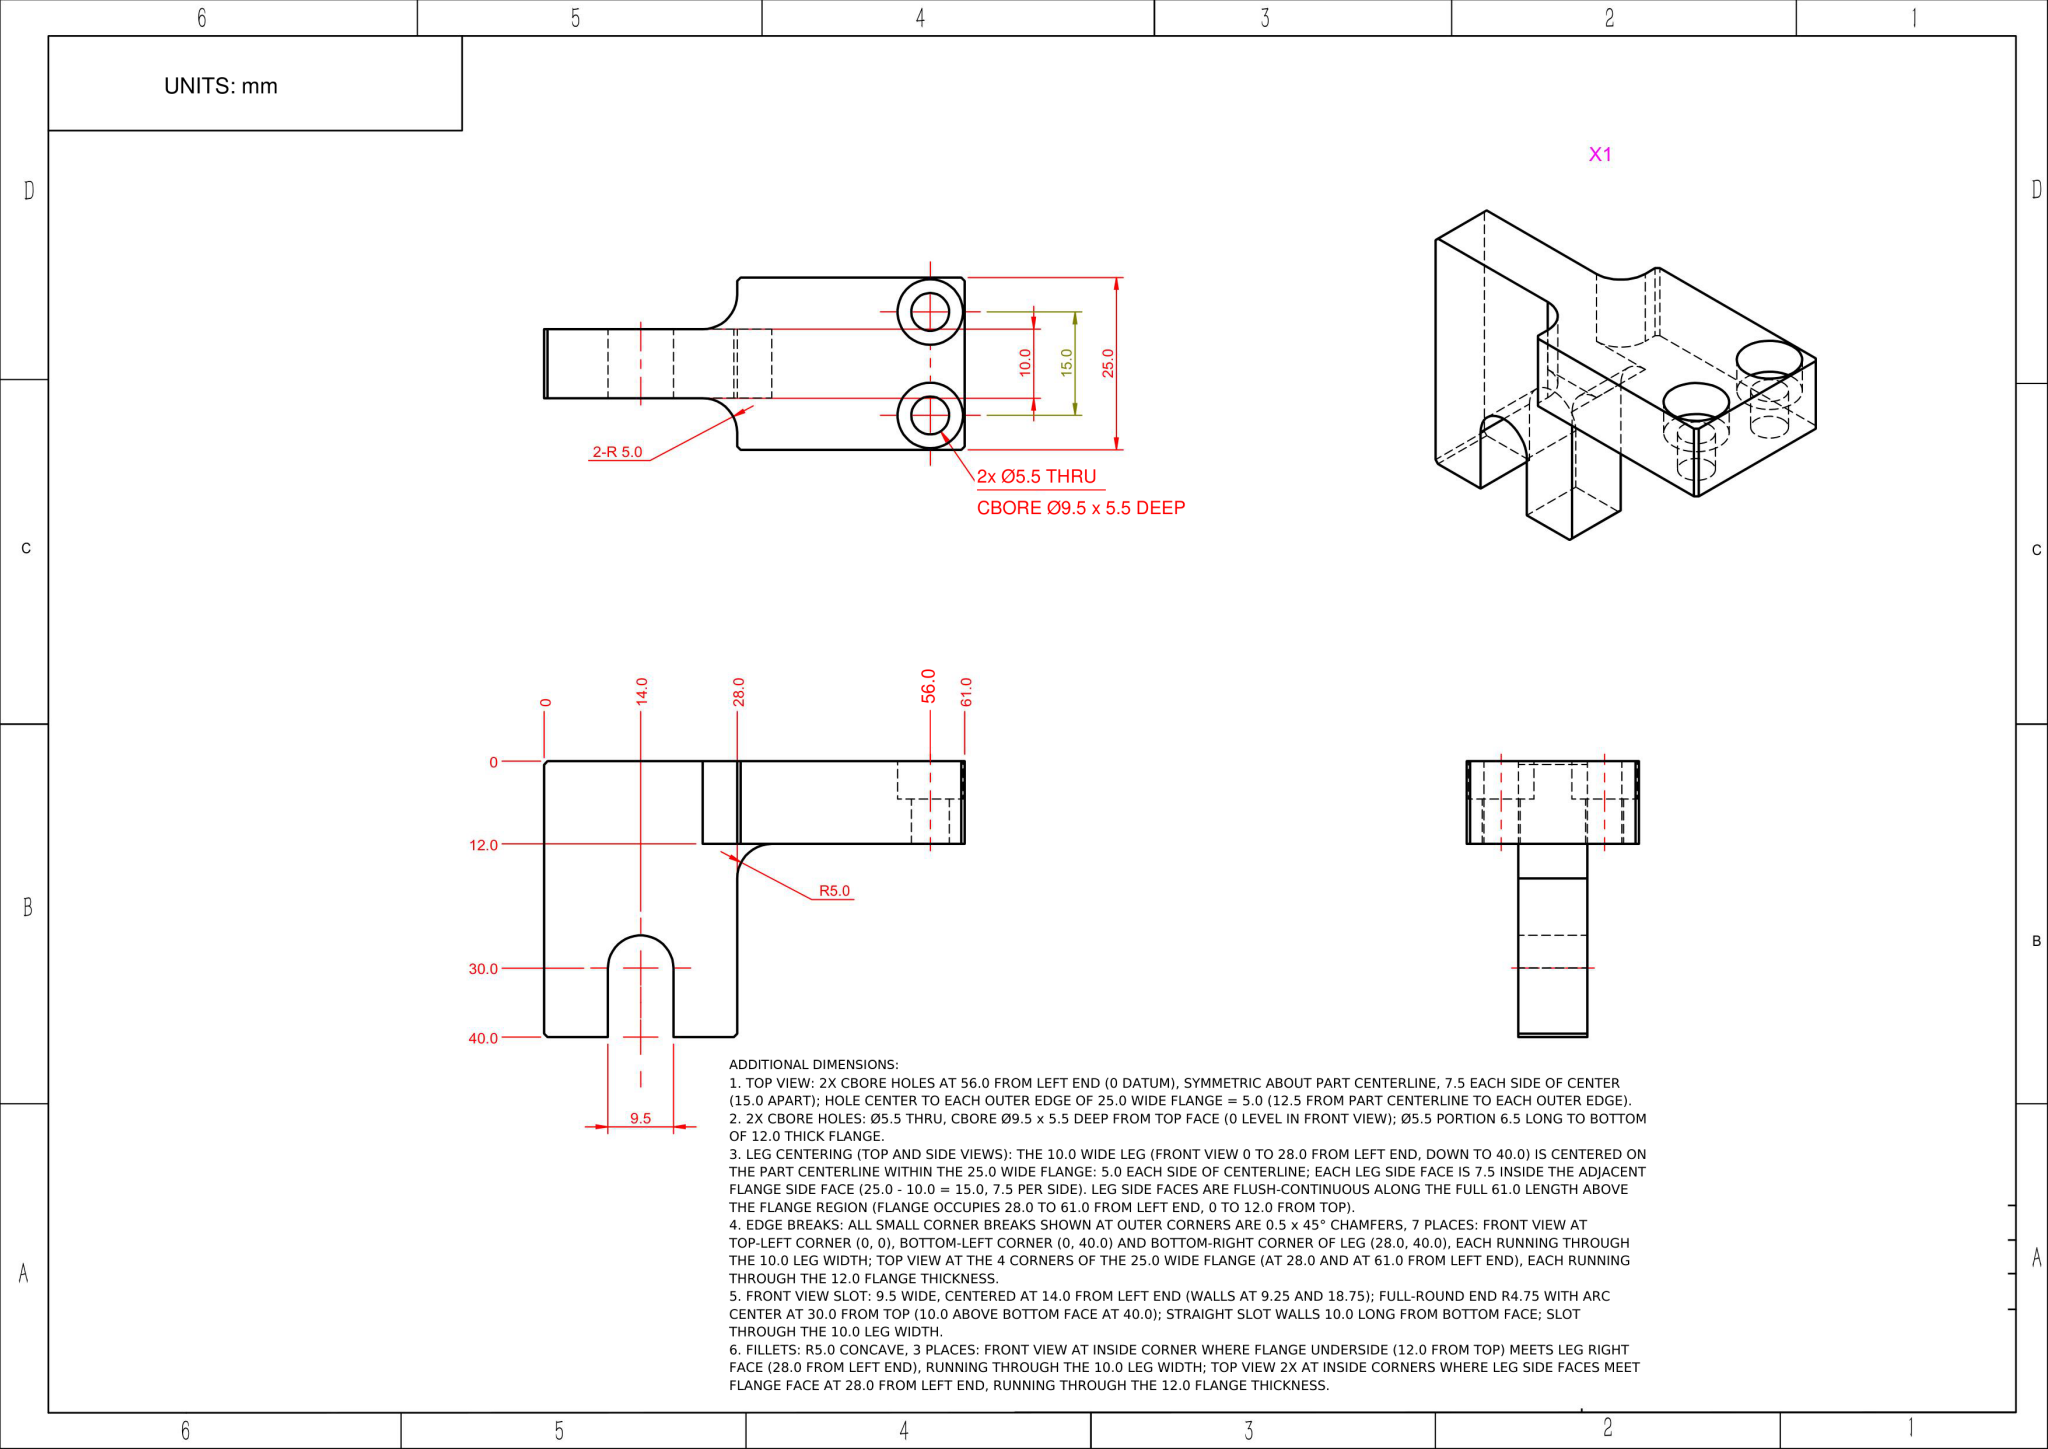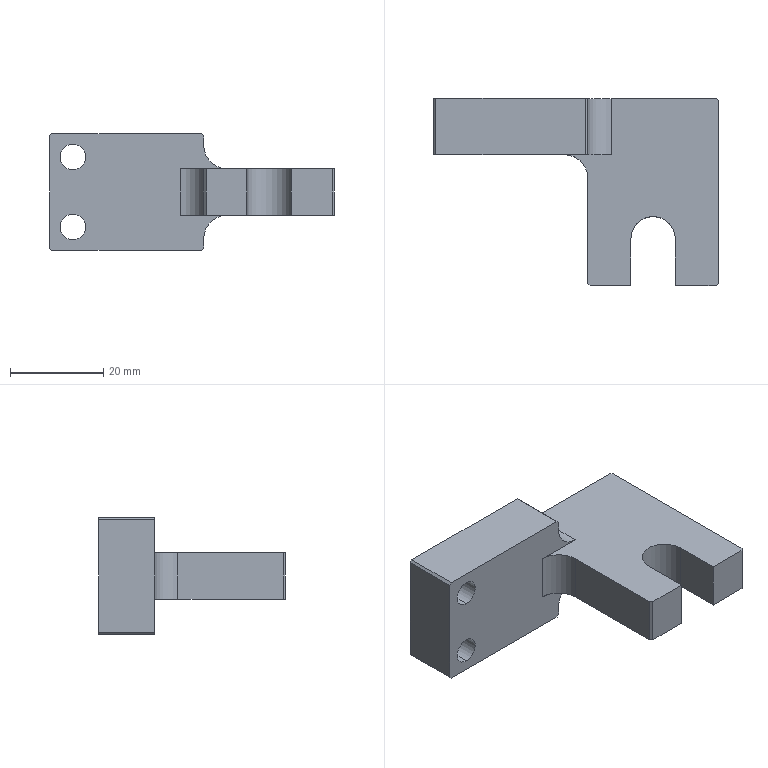Part | NX | mm | 1 solid | 36 faces | box 61 x 40 x 25 mm | volume 18880 mm3 | plane 24 | cylinder 12 | commonest cylinder face diameters 9.5 x5 5.5 x4 10 x3